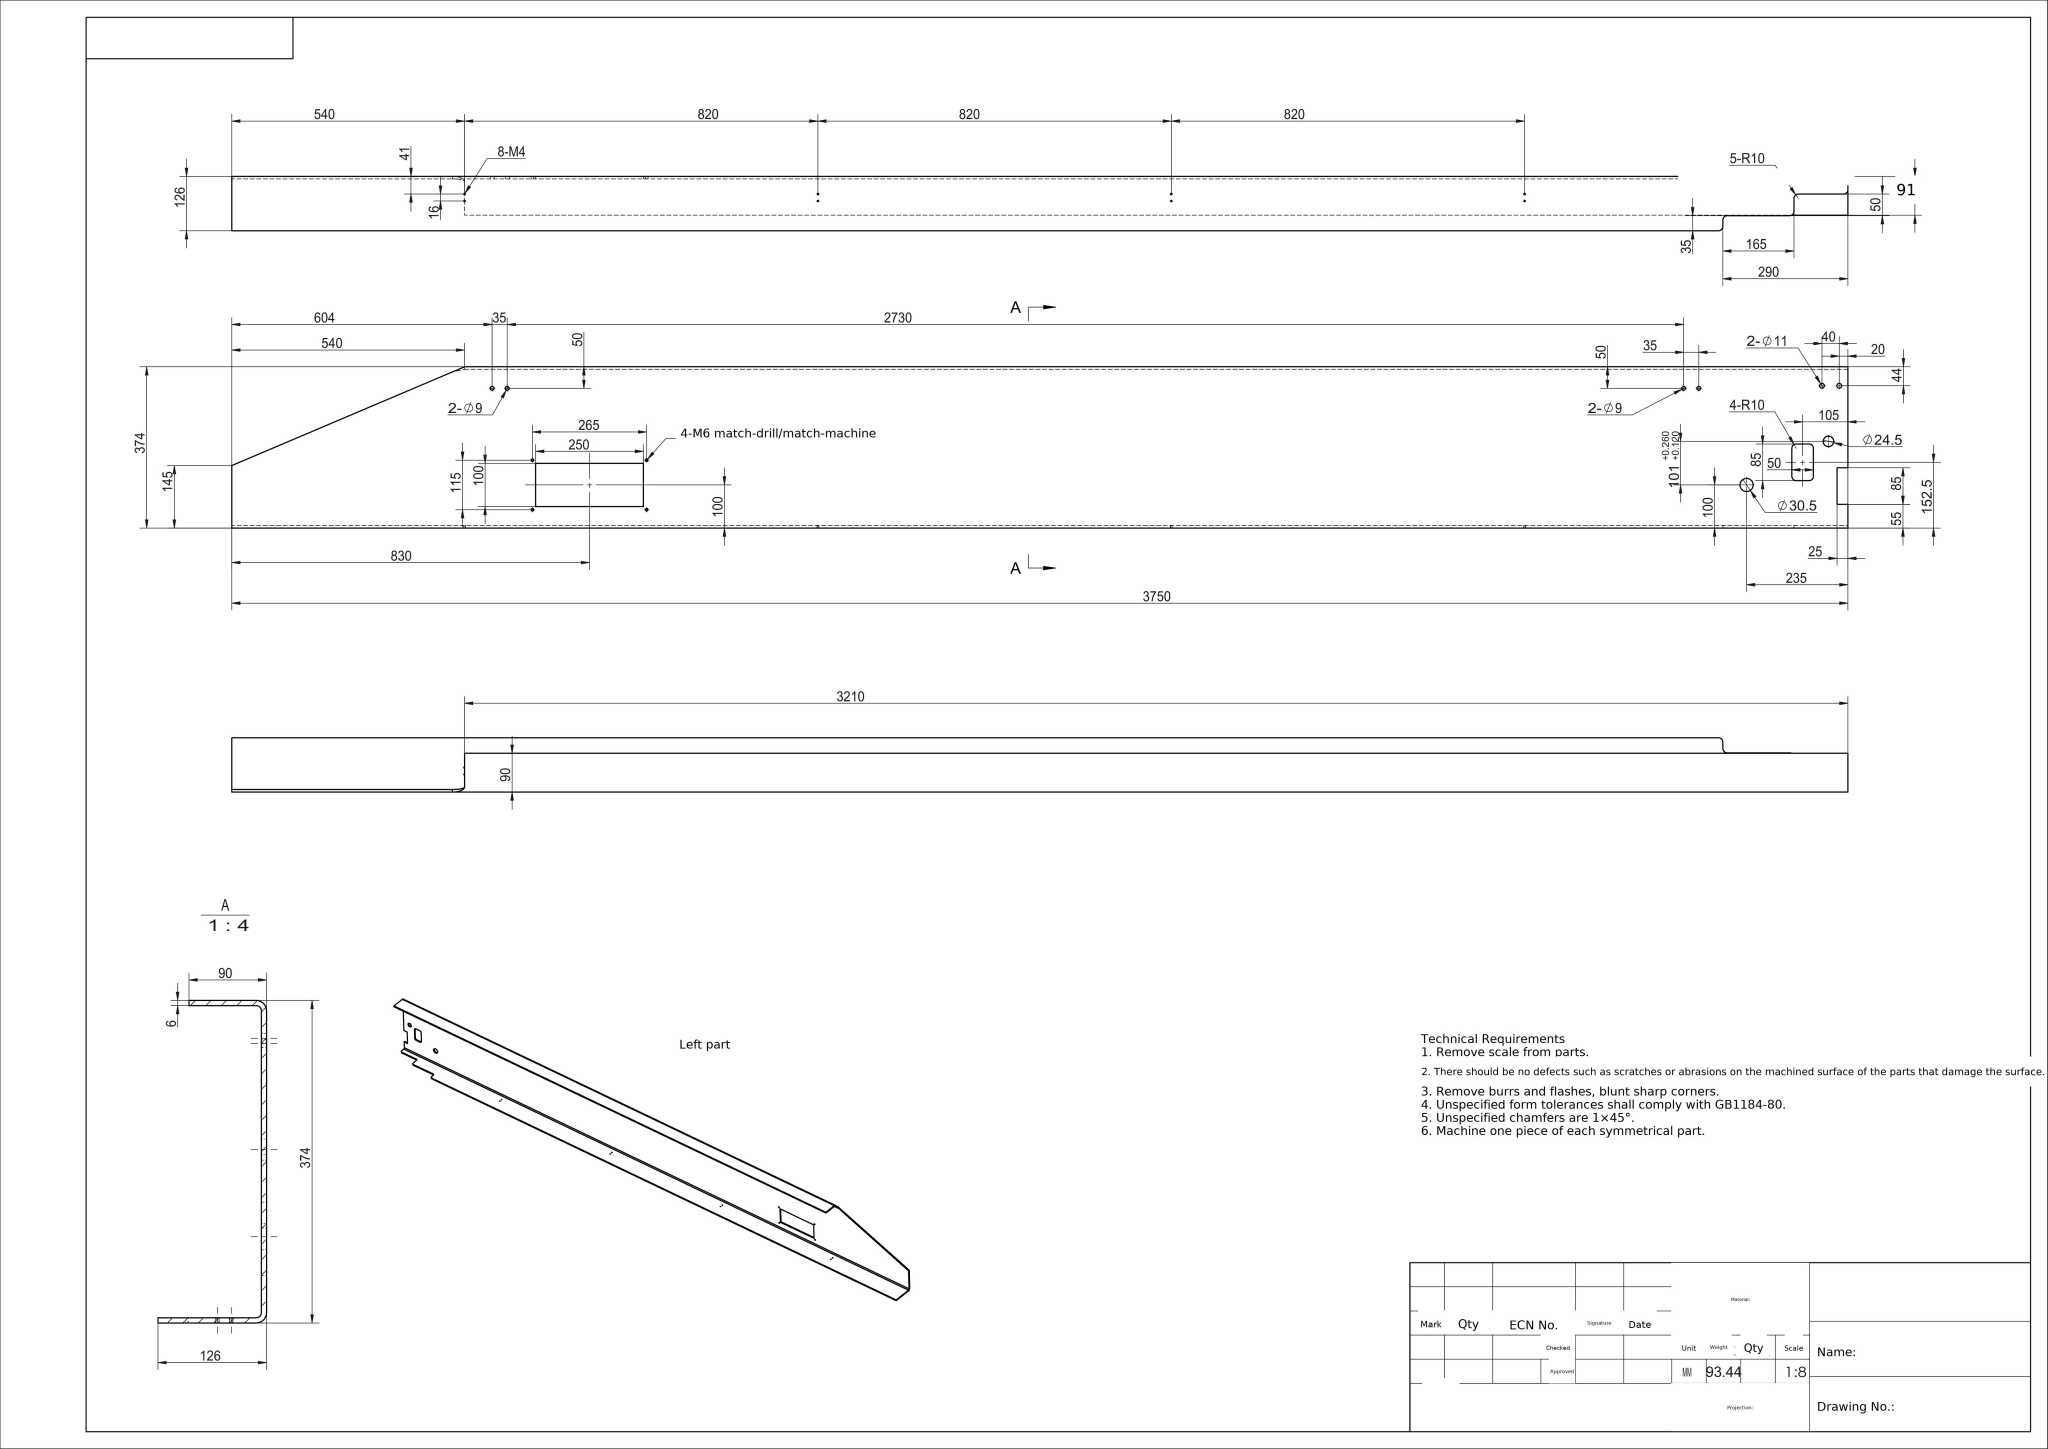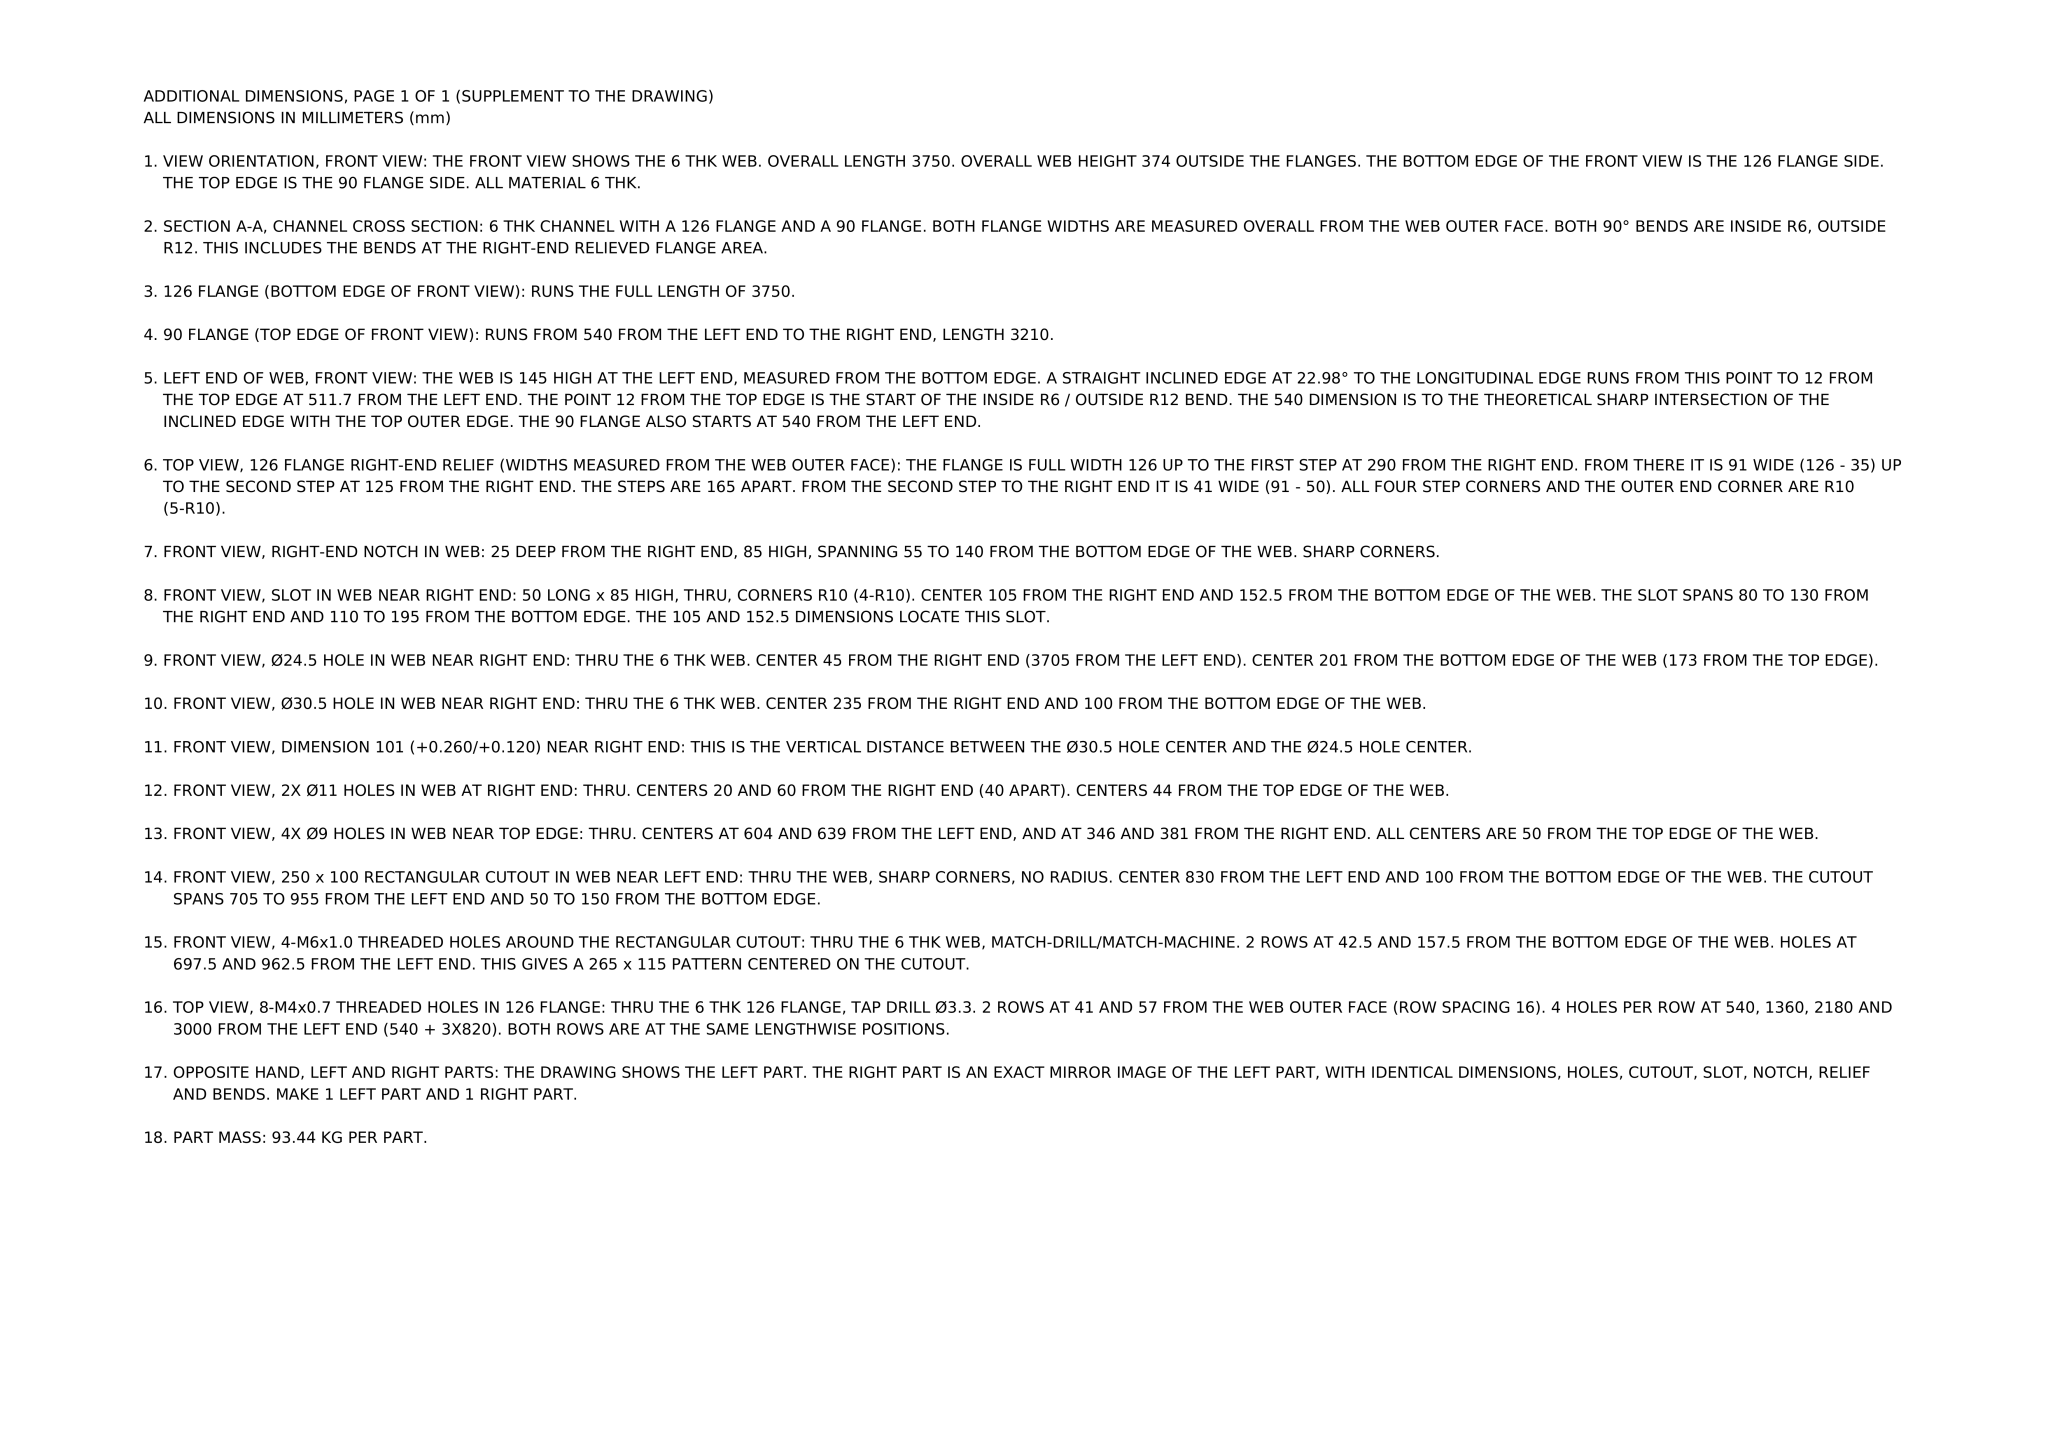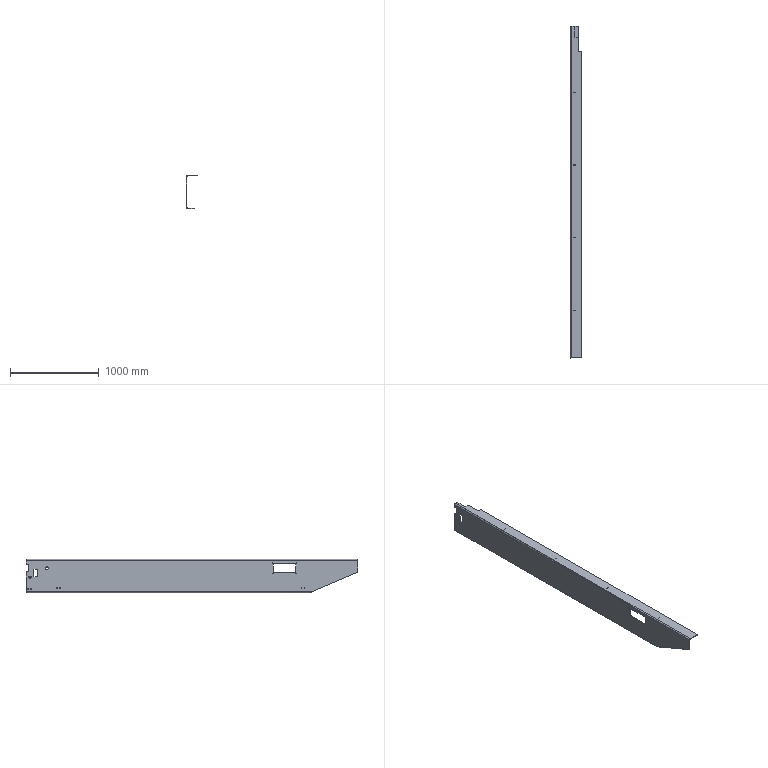Part | NX | mm | 1 solid | 88 faces | box 126 x 3750 x 374 mm | volume 11903169 mm3 | cylinder 53 | plane 34 | spline 1 | commonest cylinder face diameters 3.3 x16 20 x9 9 x8 6 x8 11 x4 30.5 x2 24.5 x2 24 x2